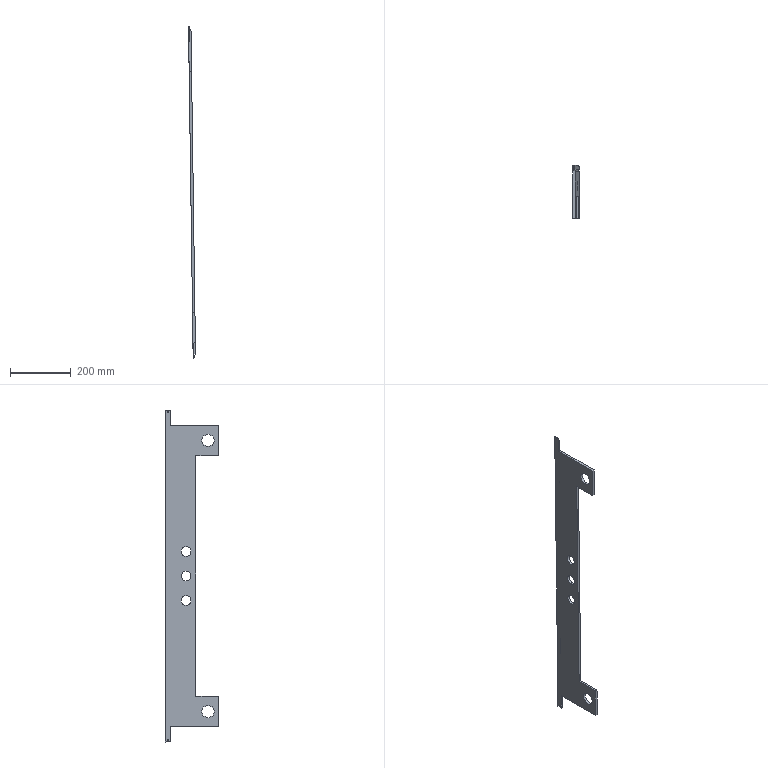Component | SolidWorks | DA-0220-Part10-10 | 1 solid | 39 faces | box 23.04 x 175 x 1089.94 mm | volume 846982 mm3 | cylinder 20 | plane 19 | commonest cylinder face diameters 19 x6 32 x6 40 x4 4.2 x4
build123d program:
from build123d import *

# Parameters (mm, degrees)
BOSS_EXTRUDE1_DEPTH         = 8
SKETCH2_W                   = 1090
SKETCH2_H                   = 2
CUT_EXTRUDE1_DEPTH          = 5
CUT_EXTRUDE2_DEPTH          = 5
CUT_EXTRUDE3_REACH          = 554.768
SKETCH7_R                   = 16
SKETCH8_W                   = 1090
SKETCH8_H                   = 2
CUT_EXTRUDE4_DEPTH          = 5
SKETCH1_3_W                 = 990
SKETCH1_3_H                 = 3
CUT_EXTRUDE1_2_DEPTH        = 5
SKETCH2_2_W                 = 100
SKETCH2_2_H                 = 75
BOSS_EXTRUDE1_2_DEPTH       = 8
SKETCH3_2_R                 = 20
CUT_EXTRUDE2_2_DEPTH        = 571.068
SKETCH1_R                   = 9.5
PULLEYCLEARANCERELIEF_DEPTH = 5


with BuildPart() as part:
    # Sketch1_2 → Boss-Extrude1 (new body)
    with BuildSketch(Plane.XY):
        Polygon((495, -8), (495, -92), (-495, -92), (-495, -8), (-545, -8), (-545, 8), (545, 8), (545, -8), align=None)
    extrude(amount=BOSS_EXTRUDE1_DEPTH)

    # Sketch2 → Cut-Extrude1 (cut)
    with BuildSketch(Plane.XY.offset(8)):
        with Locations((0, 7)):
            Rectangle(SKETCH2_W, SKETCH2_H)
    extrude(amount=-CUT_EXTRUDE1_DEPTH, mode=Mode.SUBTRACT)

    # Sketch3 → Cut-Extrude2 (cut)
    with BuildSketch(Plane.XY.offset(8)):
        with BuildLine():
            Line((-533.577, 6), (-550, 6))
            Line((-550, 6), (-550, -8))
            Line((-550, -8), (-533.577, -8))
            ThreePointArc((-533.577, -8), (-530.5, -1), (-533.577, 6))
        make_face()
    cut_extrude2 = extrude(amount=-CUT_EXTRUDE2_DEPTH, mode=Mode.SUBTRACT)

    # Sketch5 → M5 Tapped Hole1 (revolve, cut)
    with BuildSketch(Plane(origin=(-540, 0, 3), x_dir=(0, -1, 0), z_dir=(1, 0, 0))):
        Polygon((0, 0), (0, 15.262), (2.1, 14), (2.1, 0), align=None)
    m5_tapped_hole1 = revolve(axis=Axis((-540, 0, 9.35), (0, 0, -1)), mode=Mode.SUBTRACT)

    # Mirror1: Cut-Extrude2, M5 Tapped Hole1 across plane
    add(cut_extrude2.mirror(Plane(origin=(0, 0, 0), x_dir=(0, 0, 1), z_dir=(1, 0, 0))), mode=Mode.SUBTRACT)
    add(m5_tapped_hole1.mirror(Plane(origin=(0, 0, 0), x_dir=(0, 0, 1), z_dir=(1, 0, 0))), mode=Mode.SUBTRACT)

    # Sketch7 → Cut-Extrude3 (cut, up to next)
    with BuildSketch(Plane.XY.offset(8), mode=Mode.PRIVATE) as cut_extrude3_sk1:
        with Locations((0, -60)):
            Circle(SKETCH7_R)
    cut_extrude3_tool1 = extrude(cut_extrude3_sk1.sketch, amount=-CUT_EXTRUDE3_REACH, mode=Mode.PRIVATE) & part.part
    # Sketch7 → Cut-Extrude3 (cut, up to next)
    with BuildSketch(Plane.XY.offset(8), mode=Mode.PRIVATE) as cut_extrude3_sk2:
        with Locations((80, -60)):
            Circle(SKETCH7_R)
    cut_extrude3_tool2 = extrude(cut_extrude3_sk2.sketch, amount=-CUT_EXTRUDE3_REACH, mode=Mode.PRIVATE) & part.part
    # Sketch7 → Cut-Extrude3 (cut, up to next)
    with BuildSketch(Plane.XY.offset(8), mode=Mode.PRIVATE) as cut_extrude3_sk3:
        with Locations((-80, -60)):
            Circle(SKETCH7_R)
    cut_extrude3_tool3 = extrude(cut_extrude3_sk3.sketch, amount=-CUT_EXTRUDE3_REACH, mode=Mode.PRIVATE) & part.part
    add(cut_extrude3_tool1.solids().sort_by_distance((0, -60, 8))[0], mode=Mode.SUBTRACT)
    add(cut_extrude3_tool2.solids().sort_by_distance((80, -60, 8))[0], mode=Mode.SUBTRACT)
    add(cut_extrude3_tool3.solids().sort_by_distance((-80, -60, 8))[0], mode=Mode.SUBTRACT)

    # Sketch8 → Cut-Extrude4 (cut)
    with BuildSketch(Plane.XY.offset(8)):
        with Locations((0, -7)):
            Rectangle(SKETCH8_W, SKETCH8_H)
    extrude(amount=-CUT_EXTRUDE4_DEPTH, mode=Mode.SUBTRACT)

    # Sketch1_3 → Cut-Extrude1_2 (cut)
    with BuildSketch(Plane.XY.offset(8)):
        with Locations((0, -9.5)):
            Rectangle(SKETCH1_3_W, SKETCH1_3_H)
    extrude(amount=-CUT_EXTRUDE1_2_DEPTH, mode=Mode.SUBTRACT)

    # Sketch2_2 → Boss-Extrude1_2 (add)
    with BuildSketch(Plane.XY.offset(8)):
        with Locations((-445, -129.5)):
            Rectangle(SKETCH2_2_W, SKETCH2_2_H)
        with Locations((445, -129.5)):
            Rectangle(SKETCH2_2_W, SKETCH2_2_H)
    extrude(amount=-BOSS_EXTRUDE1_2_DEPTH)

    # Sketch3_2 → Cut-Extrude2_2 (cut, through all)
    with BuildSketch(Plane.XY.offset(8)):
        with Locations((-445, -132)):
            Circle(SKETCH3_2_R)
        with Locations((445, -132)):
            Circle(SKETCH3_2_R)
    extrude(amount=-CUT_EXTRUDE2_2_DEPTH, mode=Mode.SUBTRACT)

    # Sketch1 → PulleyClearanceRelief (cut)
    with BuildSketch(Plane.XY.offset(8)):
        with Locations((-540, 0)):
            Circle(SKETCH1_R)
        with Locations((540, 0)):
            Circle(SKETCH1_R)
    extrude(amount=-PULLEYCLEARANCERELIEF_DEPTH, mode=Mode.SUBTRACT)


solid = part.part

# Placed as in the assembly
solid = solid.moved(Location((496.107, -33.852, 10.424), (-1.659, 89.2, 1.659)))